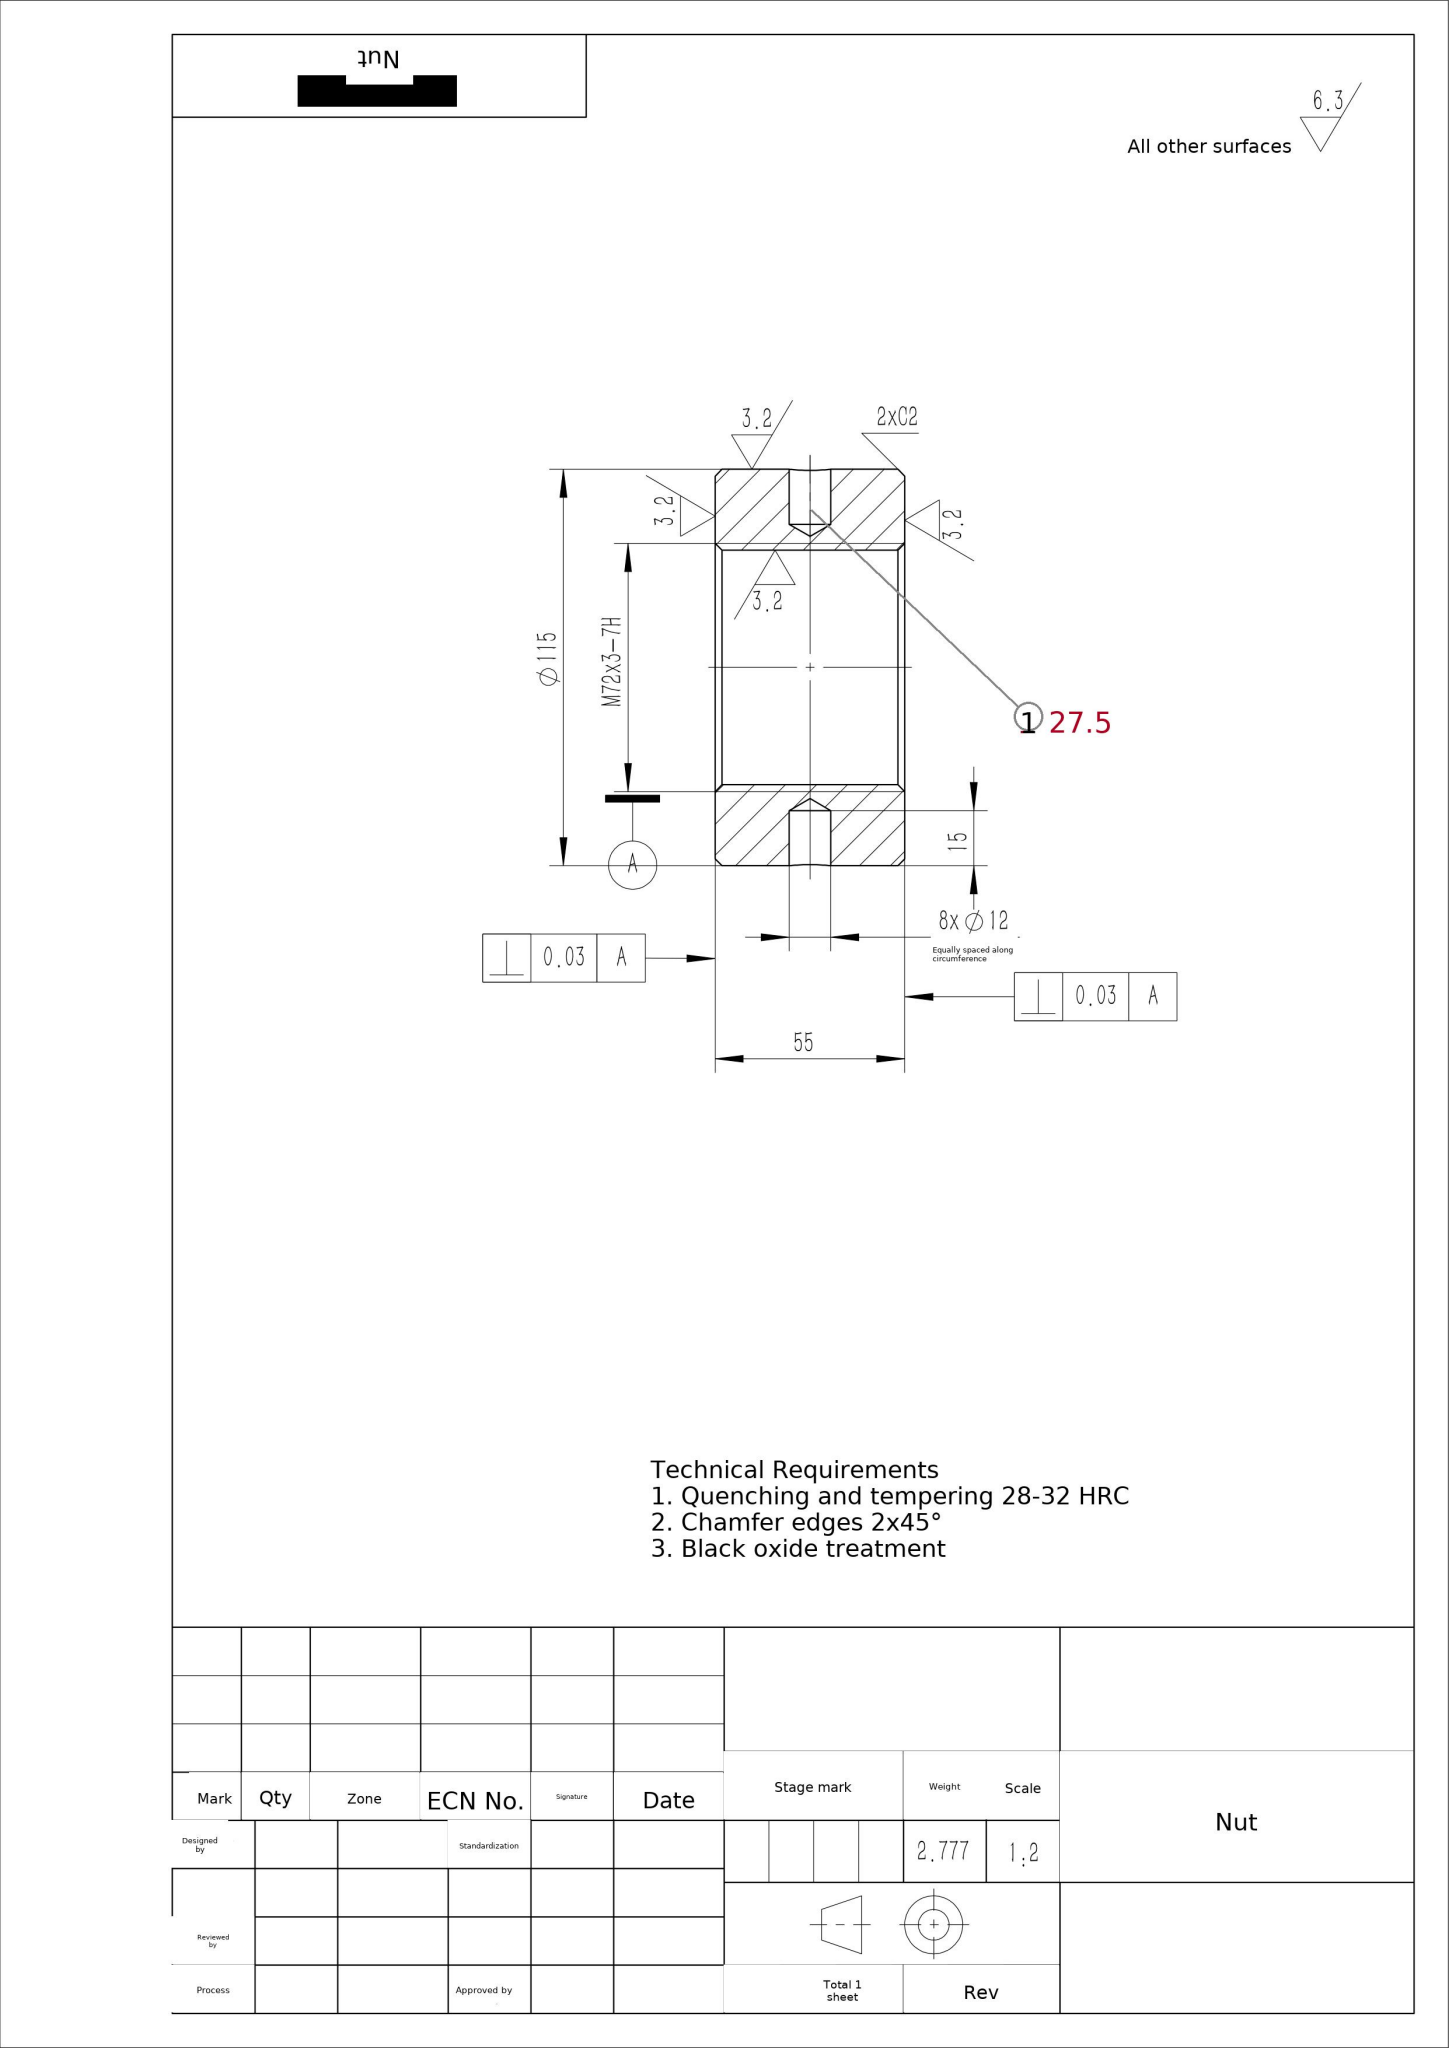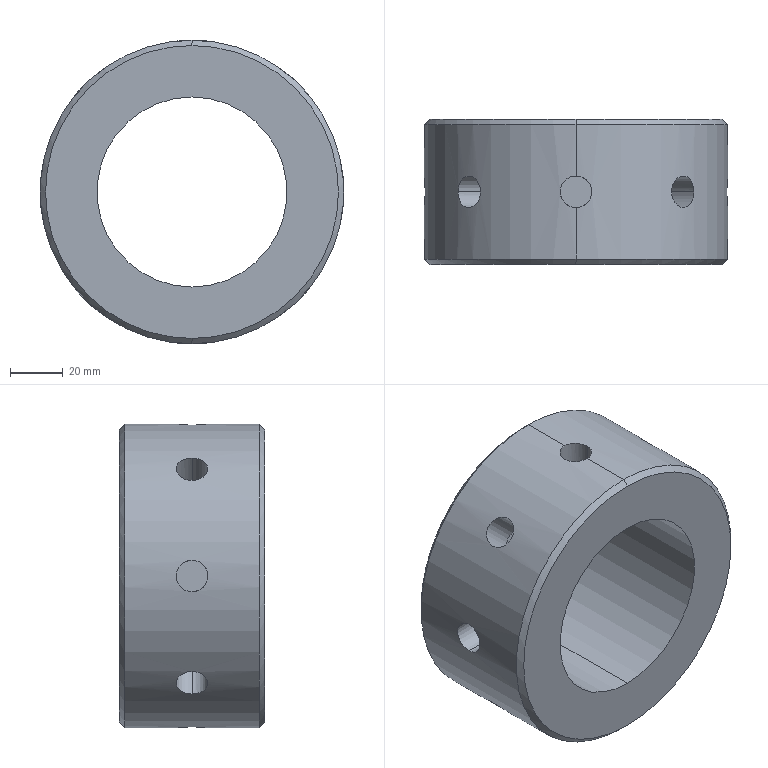Part | SolidWorks | mm | 1 solid | 34 faces | box 115 x 55 x 115 mm | volume 332415 mm3 | cylinder 20 | plane 10 | cone 4 | commonest cylinder face diameters 12 x16 72 x2 115 x2
build123d program:
from build123d import *

# Parameters (mm, degrees)
SKETCH1_R           = 57.5
SKETCH1_R_2         = 36
BOSS_EXTRUDE2_DEPTH = 55
CHAMFER1_SIZE       = 2
CUT_EXTRUDE2_START  = 57.5
SKETCH6_R           = 6
CUT_EXTRUDE2_DEPTH  = 15
CIRPATTERN1_COUNT   = 8


with BuildPart() as part:
    # Sketch1 → Boss-Extrude2 (new body)
    with BuildSketch(Plane(origin=(0, 0, 0), x_dir=(1, 0, 0), z_dir=(0, 1, 0))):
        with Locations(Location((0, 0, 0), (0, 0, 270))):
            Circle(SKETCH1_R)
        with Locations(Location((0, 0, 0), (0, 0, 270))):
            Circle(SKETCH1_R_2, mode=Mode.SUBTRACT)
    extrude(amount=BOSS_EXTRUDE2_DEPTH)

    # Chamfer1
    chamfer1_edges = [part.edges().sort_by_distance(p)[0] for p in [
        (0, 0, -57.5),
        (0, 55, -57.5),
    ]]
    chamfer(chamfer1_edges, length=CHAMFER1_SIZE)

    # Sketch6 → Cut-Extrude2 (cut)
    with BuildSketch(Plane.XY.offset(CUT_EXTRUDE2_START)):
        with Locations((0, 27.5)):
            Circle(SKETCH6_R)
    cut_extrude2 = extrude(amount=-CUT_EXTRUDE2_DEPTH, mode=Mode.SUBTRACT)

    # CirPattern1: Cut-Extrude2 ×8 about axis
    cirpattern1_axis = Axis((0, 0, 0), (0, 1, 0))
    for i in range(1, CIRPATTERN1_COUNT):
        add(cut_extrude2.rotate(cirpattern1_axis, i * 360 / CIRPATTERN1_COUNT), mode=Mode.SUBTRACT)


solid = part.part